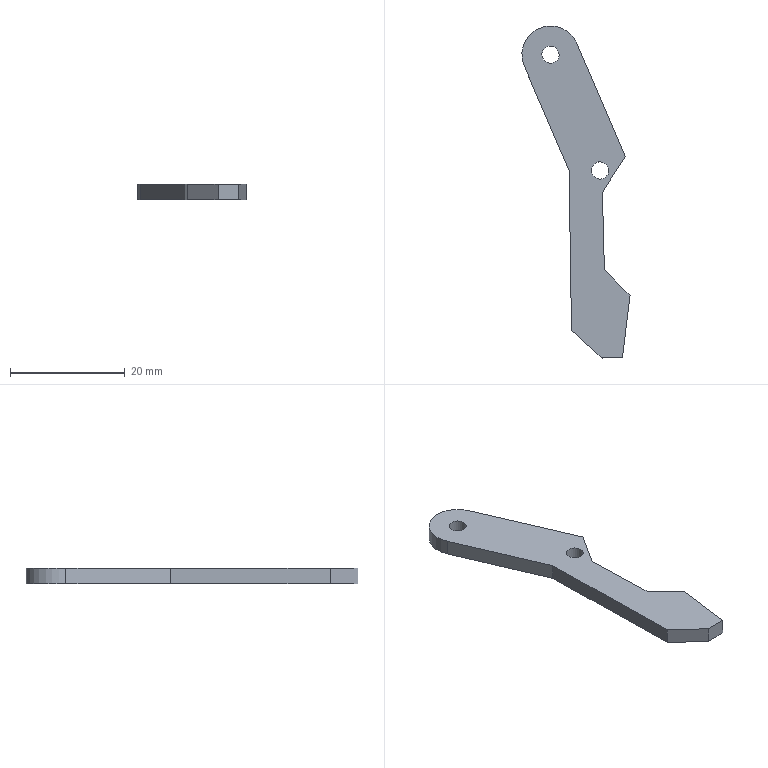Component | NX | GRIPPER_3 | 1 solid | 14 faces | box 18.88 x 57.93 x 2.7 mm | volume 1283 mm3 | plane 11 | cylinder 3 | commonest cylinder face diameters 3 x2 10 x1
STEP:
#1=CARTESIAN_POINT('',(0.,0.,0.));
#2=DIRECTION('',(0.,0.,1.));
#3=DIRECTION('',(1.,0.,0.));
#4=AXIS2_PLACEMENT_3D('',#1,#2,#3);
#5=CARTESIAN_POINT('',(-5.132,-91.783,35.05));
#6=VERTEX_POINT('',#5);
#7=CARTESIAN_POINT('',(-8.684,-91.838,35.05));
#8=VERTEX_POINT('',#7);
#9=CARTESIAN_POINT('',(-5.132,-91.783,35.05));
#10=DIRECTION('',(-0.9999,-0.01539,0.));
#11=VECTOR('',#10,1.);
#12=LINE('',#9,#11);
#13=CARTESIAN_POINT('',(-5.132,-91.783,32.35));
#14=DIRECTION('',(-0.01539,0.9999,0.));
#15=DIRECTION('',(-0.9999,-0.01539,0.));
#16=AXIS2_PLACEMENT_3D('',#13,#14,#15);
#17=PLANE('',#16);
#18=CARTESIAN_POINT('',(0.,2.7));
#19=DIRECTION('',(1.,0.));
#20=VECTOR('',#19,1.);
#21=LINE('',#18,#20);
#22=(GEOMETRIC_REPRESENTATION_CONTEXT(2)PARAMETRIC_REPRESENTATION_CONTEXT()REPRESENTATION_CONTEXT('',''));
#23=DEFINITIONAL_REPRESENTATION('',(#21),#22);
#24=PCURVE('',#17,#23);
#25=CARTESIAN_POINT('',(-17.683,-38.904,35.05));
#26=DIRECTION('',(0.,0.,-1.));
#27=DIRECTION('',(0.9189,0.3945,0.));
#28=AXIS2_PLACEMENT_3D('',#25,#26,#27);
#29=PLANE('',#28);
#30=CARTESIAN_POINT('',(-9.325,53.542));
#31=DIRECTION('',(-0.9249,-0.3803));
#32=VECTOR('',#31,1.);
#33=LINE('',#30,#32);
#34=(GEOMETRIC_REPRESENTATION_CONTEXT(2)PARAMETRIC_REPRESENTATION_CONTEXT()REPRESENTATION_CONTEXT('',''));
#35=DEFINITIONAL_REPRESENTATION('',(#33),#34);
#36=PCURVE('',#29,#35);
#37=SURFACE_CURVE('',#12,(#24,#36),.PCURVE_S1.);
#38=EDGE_CURVE('',#6,#8,#37,.T.);
#39=ORIENTED_EDGE('',*,*,#38,.T.);
#40=CARTESIAN_POINT('',(-8.684,-91.838,32.35));
#41=VERTEX_POINT('',#40);
#42=CARTESIAN_POINT('',(-8.684,-91.838,32.35));
#43=DIRECTION('',(0.,0.,1.));
#44=VECTOR('',#43,1.);
#45=LINE('',#42,#44);
#46=CARTESIAN_POINT('',(3.552,0.));
#47=DIRECTION('',(0.,1.));
#48=VECTOR('',#47,1.);
#49=LINE('',#46,#48);
#50=(GEOMETRIC_REPRESENTATION_CONTEXT(2)PARAMETRIC_REPRESENTATION_CONTEXT()REPRESENTATION_CONTEXT('',''));
#51=DEFINITIONAL_REPRESENTATION('',(#49),#50);
#52=PCURVE('',#17,#51);
#53=CARTESIAN_POINT('',(-8.684,-91.838,32.35));
#54=DIRECTION('',(0.6727,0.7399,0.));
#55=DIRECTION('',(-0.7399,0.6727,0.));
#56=AXIS2_PLACEMENT_3D('',#53,#54,#55);
#57=PLANE('',#56);
#58=CARTESIAN_POINT('',(0.,0.));
#59=DIRECTION('',(0.,1.));
#60=VECTOR('',#59,1.);
#61=LINE('',#58,#60);
#62=(GEOMETRIC_REPRESENTATION_CONTEXT(2)PARAMETRIC_REPRESENTATION_CONTEXT()REPRESENTATION_CONTEXT('',''));
#63=DEFINITIONAL_REPRESENTATION('',(#61),#62);
#64=PCURVE('',#57,#63);
#65=SURFACE_CURVE('',#45,(#52,#64),.PCURVE_S1.);
#66=EDGE_CURVE('',#41,#8,#65,.T.);
#67=ORIENTED_EDGE('',*,*,#66,.F.);
#68=CARTESIAN_POINT('',(-5.132,-91.783,32.35));
#69=VERTEX_POINT('',#68);
#70=CARTESIAN_POINT('',(-5.132,-91.783,32.35));
#71=DIRECTION('',(-0.9999,-0.01539,0.));
#72=VECTOR('',#71,1.);
#73=LINE('',#70,#72);
#74=CARTESIAN_POINT('',(0.,0.));
#75=DIRECTION('',(1.,0.));
#76=VECTOR('',#75,1.);
#77=LINE('',#74,#76);
#78=(GEOMETRIC_REPRESENTATION_CONTEXT(2)PARAMETRIC_REPRESENTATION_CONTEXT()REPRESENTATION_CONTEXT('',''));
#79=DEFINITIONAL_REPRESENTATION('',(#77),#78);
#80=PCURVE('',#17,#79);
#81=CARTESIAN_POINT('',(-17.683,-38.904,32.35));
#82=DIRECTION('',(0.,0.,-1.));
#83=DIRECTION('',(0.9189,0.3945,0.));
#84=AXIS2_PLACEMENT_3D('',#81,#82,#83);
#85=PLANE('',#84);
#86=CARTESIAN_POINT('',(-9.325,53.542));
#87=DIRECTION('',(-0.9249,-0.3803));
#88=VECTOR('',#87,1.);
#89=LINE('',#86,#88);
#90=(GEOMETRIC_REPRESENTATION_CONTEXT(2)PARAMETRIC_REPRESENTATION_CONTEXT()REPRESENTATION_CONTEXT('',''));
#91=DEFINITIONAL_REPRESENTATION('',(#89),#90);
#92=PCURVE('',#85,#91);
#93=SURFACE_CURVE('',#73,(#80,#92),.PCURVE_S1.);
#94=EDGE_CURVE('',#69,#41,#93,.T.);
#95=ORIENTED_EDGE('',*,*,#94,.F.);
#96=CARTESIAN_POINT('',(-5.132,-91.783,32.35));
#97=DIRECTION('',(0.,0.,1.));
#98=VECTOR('',#97,1.);
#99=LINE('',#96,#98);
#100=CARTESIAN_POINT('',(0.,0.));
#101=DIRECTION('',(0.,1.));
#102=VECTOR('',#101,1.);
#103=LINE('',#100,#102);
#104=(GEOMETRIC_REPRESENTATION_CONTEXT(2)PARAMETRIC_REPRESENTATION_CONTEXT()REPRESENTATION_CONTEXT('',''));
#105=DEFINITIONAL_REPRESENTATION('',(#103),#104);
#106=PCURVE('',#17,#105);
#107=CARTESIAN_POINT('',(-3.8,-80.896,32.35));
#108=DIRECTION('',(-0.9926,0.1214,0.));
#109=DIRECTION('',(-0.1214,-0.9926,0.));
#110=AXIS2_PLACEMENT_3D('',#107,#108,#109);
#111=PLANE('',#110);
#112=CARTESIAN_POINT('',(10.969,0.));
#113=DIRECTION('',(0.,1.));
#114=VECTOR('',#113,1.);
#115=LINE('',#112,#114);
#116=(GEOMETRIC_REPRESENTATION_CONTEXT(2)PARAMETRIC_REPRESENTATION_CONTEXT()REPRESENTATION_CONTEXT('',''));
#117=DEFINITIONAL_REPRESENTATION('',(#115),#116);
#118=PCURVE('',#111,#117);
#119=SURFACE_CURVE('',#99,(#106,#118),.PCURVE_S1.);
#120=EDGE_CURVE('',#69,#6,#119,.T.);
#121=ORIENTED_EDGE('',*,*,#120,.T.);
#122=EDGE_LOOP('',(#39,#67,#95,#121));
#123=FACE_BOUND('',#122,.T.);
#124=ADVANCED_FACE('',(#123),#17,.F.);
#125=CARTESIAN_POINT('',(-14.019,-86.988,35.05));
#126=VERTEX_POINT('',#125);
#127=CARTESIAN_POINT('',(-8.684,-91.838,35.05));
#128=DIRECTION('',(-0.7399,0.6727,0.));
#129=VECTOR('',#128,1.);
#130=LINE('',#127,#129);
#131=CARTESIAN_POINT('',(0.,2.7));
#132=DIRECTION('',(1.,0.));
#133=VECTOR('',#132,1.);
#134=LINE('',#131,#133);
#135=(GEOMETRIC_REPRESENTATION_CONTEXT(2)PARAMETRIC_REPRESENTATION_CONTEXT()REPRESENTATION_CONTEXT('',''));
#136=DEFINITIONAL_REPRESENTATION('',(#134),#135);
#137=PCURVE('',#57,#136);
#138=CARTESIAN_POINT('',(-12.611,52.191));
#139=DIRECTION('',(-0.4145,-0.91));
#140=VECTOR('',#139,1.);
#141=LINE('',#138,#140);
#142=(GEOMETRIC_REPRESENTATION_CONTEXT(2)PARAMETRIC_REPRESENTATION_CONTEXT()REPRESENTATION_CONTEXT('',''));
#143=DEFINITIONAL_REPRESENTATION('',(#141),#142);
#144=PCURVE('',#29,#143);
#145=SURFACE_CURVE('',#130,(#137,#144),.PCURVE_S1.);
#146=EDGE_CURVE('',#8,#126,#145,.T.);
#147=ORIENTED_EDGE('',*,*,#146,.T.);
#148=CARTESIAN_POINT('',(-14.019,-86.988,32.35));
#149=VERTEX_POINT('',#148);
#150=CARTESIAN_POINT('',(-14.019,-86.988,32.35));
#151=DIRECTION('',(0.,0.,1.));
#152=VECTOR('',#151,1.);
#153=LINE('',#150,#152);
#154=CARTESIAN_POINT('',(7.21,0.));
#155=DIRECTION('',(0.,1.));
#156=VECTOR('',#155,1.);
#157=LINE('',#154,#156);
#158=(GEOMETRIC_REPRESENTATION_CONTEXT(2)PARAMETRIC_REPRESENTATION_CONTEXT()REPRESENTATION_CONTEXT('',''));
#159=DEFINITIONAL_REPRESENTATION('',(#157),#158);
#160=PCURVE('',#57,#159);
#161=CARTESIAN_POINT('',(-14.019,-86.988,32.35));
#162=DIRECTION('',(0.9999,0.01539,0.));
#163=DIRECTION('',(-0.01539,0.9999,0.));
#164=AXIS2_PLACEMENT_3D('',#161,#162,#163);
#165=PLANE('',#164);
#166=CARTESIAN_POINT('',(0.,0.));
#167=DIRECTION('',(0.,1.));
#168=VECTOR('',#167,1.);
#169=LINE('',#166,#168);
#170=(GEOMETRIC_REPRESENTATION_CONTEXT(2)PARAMETRIC_REPRESENTATION_CONTEXT()REPRESENTATION_CONTEXT('',''));
#171=DEFINITIONAL_REPRESENTATION('',(#169),#170);
#172=PCURVE('',#165,#171);
#173=SURFACE_CURVE('',#153,(#160,#172),.PCURVE_S1.);
#174=EDGE_CURVE('',#149,#126,#173,.T.);
#175=ORIENTED_EDGE('',*,*,#174,.F.);
#176=CARTESIAN_POINT('',(-8.684,-91.838,32.35));
#177=DIRECTION('',(-0.7399,0.6727,0.));
#178=VECTOR('',#177,1.);
#179=LINE('',#176,#178);
#180=CARTESIAN_POINT('',(0.,0.));
#181=DIRECTION('',(1.,0.));
#182=VECTOR('',#181,1.);
#183=LINE('',#180,#182);
#184=(GEOMETRIC_REPRESENTATION_CONTEXT(2)PARAMETRIC_REPRESENTATION_CONTEXT()REPRESENTATION_CONTEXT('',''));
#185=DEFINITIONAL_REPRESENTATION('',(#183),#184);
#186=PCURVE('',#57,#185);
#187=CARTESIAN_POINT('',(-12.611,52.191));
#188=DIRECTION('',(-0.4145,-0.91));
#189=VECTOR('',#188,1.);
#190=LINE('',#187,#189);
#191=(GEOMETRIC_REPRESENTATION_CONTEXT(2)PARAMETRIC_REPRESENTATION_CONTEXT()REPRESENTATION_CONTEXT('',''));
#192=DEFINITIONAL_REPRESENTATION('',(#190),#191);
#193=PCURVE('',#85,#192);
#194=SURFACE_CURVE('',#179,(#186,#193),.PCURVE_S1.);
#195=EDGE_CURVE('',#41,#149,#194,.T.);
#196=ORIENTED_EDGE('',*,*,#195,.F.);
#197=ORIENTED_EDGE('',*,*,#66,.T.);
#198=EDGE_LOOP('',(#147,#175,#196,#197));
#199=FACE_BOUND('',#198,.T.);
#200=ADVANCED_FACE('',(#199),#57,.F.);
#201=CARTESIAN_POINT('',(-14.448,-59.117,35.05));
#202=VERTEX_POINT('',#201);
#203=CARTESIAN_POINT('',(-14.019,-86.988,35.05));
#204=DIRECTION('',(-0.01539,0.9999,0.));
#205=VECTOR('',#204,1.);
#206=LINE('',#203,#205);
#207=CARTESIAN_POINT('',(0.,2.7));
#208=DIRECTION('',(1.,0.));
#209=VECTOR('',#208,1.);
#210=LINE('',#207,#209);
#211=(GEOMETRIC_REPRESENTATION_CONTEXT(2)PARAMETRIC_REPRESENTATION_CONTEXT()REPRESENTATION_CONTEXT('',''));
#212=DEFINITIONAL_REPRESENTATION('',(#210),#211);
#213=PCURVE('',#165,#212);
#214=CARTESIAN_POINT('',(-15.599,45.63));
#215=DIRECTION('',(0.3803,-0.9249));
#216=VECTOR('',#215,1.);
#217=LINE('',#214,#216);
#218=(GEOMETRIC_REPRESENTATION_CONTEXT(2)PARAMETRIC_REPRESENTATION_CONTEXT()REPRESENTATION_CONTEXT('',''));
#219=DEFINITIONAL_REPRESENTATION('',(#217),#218);
#220=PCURVE('',#29,#219);
#221=SURFACE_CURVE('',#206,(#213,#220),.PCURVE_S1.);
#222=EDGE_CURVE('',#126,#202,#221,.T.);
#223=ORIENTED_EDGE('',*,*,#222,.T.);
#224=CARTESIAN_POINT('',(-14.448,-59.117,32.35));
#225=VERTEX_POINT('',#224);
#226=CARTESIAN_POINT('',(-14.448,-59.117,32.35));
#227=DIRECTION('',(0.,0.,1.));
#228=VECTOR('',#227,1.);
#229=LINE('',#226,#228);
#230=CARTESIAN_POINT('',(27.874,0.));
#231=DIRECTION('',(0.,1.));
#232=VECTOR('',#231,1.);
#233=LINE('',#230,#232);
#234=(GEOMETRIC_REPRESENTATION_CONTEXT(2)PARAMETRIC_REPRESENTATION_CONTEXT()REPRESENTATION_CONTEXT('',''));
#235=DEFINITIONAL_REPRESENTATION('',(#233),#234);
#236=PCURVE('',#165,#235);
#237=CARTESIAN_POINT('',(-14.448,-59.117,32.35));
#238=DIRECTION('',(0.9189,0.3945,0.));
#239=DIRECTION('',(-0.3945,0.9189,0.));
#240=AXIS2_PLACEMENT_3D('',#237,#238,#239);
#241=PLANE('',#240);
#242=CARTESIAN_POINT('',(0.,0.));
#243=DIRECTION('',(0.,1.));
#244=VECTOR('',#243,1.);
#245=LINE('',#242,#244);
#246=(GEOMETRIC_REPRESENTATION_CONTEXT(2)PARAMETRIC_REPRESENTATION_CONTEXT()REPRESENTATION_CONTEXT('',''));
#247=DEFINITIONAL_REPRESENTATION('',(#245),#246);
#248=PCURVE('',#241,#247);
#249=SURFACE_CURVE('',#229,(#236,#248),.PCURVE_S1.);
#250=EDGE_CURVE('',#225,#202,#249,.T.);
#251=ORIENTED_EDGE('',*,*,#250,.F.);
#252=CARTESIAN_POINT('',(-14.019,-86.988,32.35));
#253=DIRECTION('',(-0.01539,0.9999,0.));
#254=VECTOR('',#253,1.);
#255=LINE('',#252,#254);
#256=CARTESIAN_POINT('',(0.,0.));
#257=DIRECTION('',(1.,0.));
#258=VECTOR('',#257,1.);
#259=LINE('',#256,#258);
#260=(GEOMETRIC_REPRESENTATION_CONTEXT(2)PARAMETRIC_REPRESENTATION_CONTEXT()REPRESENTATION_CONTEXT('',''));
#261=DEFINITIONAL_REPRESENTATION('',(#259),#260);
#262=PCURVE('',#165,#261);
#263=CARTESIAN_POINT('',(-15.599,45.63));
#264=DIRECTION('',(0.3803,-0.9249));
#265=VECTOR('',#264,1.);
#266=LINE('',#263,#265);
#267=(GEOMETRIC_REPRESENTATION_CONTEXT(2)PARAMETRIC_REPRESENTATION_CONTEXT()REPRESENTATION_CONTEXT('',''));
#268=DEFINITIONAL_REPRESENTATION('',(#266),#267);
#269=PCURVE('',#85,#268);
#270=SURFACE_CURVE('',#255,(#262,#269),.PCURVE_S1.);
#271=EDGE_CURVE('',#149,#225,#270,.T.);
#272=ORIENTED_EDGE('',*,*,#271,.F.);
#273=ORIENTED_EDGE('',*,*,#174,.T.);
#274=EDGE_LOOP('',(#223,#251,#272,#273));
#275=FACE_BOUND('',#274,.T.);
#276=ADVANCED_FACE('',(#275),#165,.F.);
#277=CARTESIAN_POINT('',(-22.278,-40.877,35.05));
#278=VERTEX_POINT('',#277);
#279=CARTESIAN_POINT('',(-14.448,-59.117,35.05));
#280=DIRECTION('',(-0.3945,0.9189,0.));
#281=VECTOR('',#280,1.);
#282=LINE('',#279,#281);
#283=CARTESIAN_POINT('',(0.,2.7));
#284=DIRECTION('',(1.,0.));
#285=VECTOR('',#284,1.);
#286=LINE('',#283,#285);
#287=(GEOMETRIC_REPRESENTATION_CONTEXT(2)PARAMETRIC_REPRESENTATION_CONTEXT()REPRESENTATION_CONTEXT('',''));
#288=DEFINITIONAL_REPRESENTATION('',(#286),#287);
#289=PCURVE('',#241,#288);
#290=CARTESIAN_POINT('',(-5.,19.85));
#291=DIRECTION('',(0.,-1.));
#292=VECTOR('',#291,1.);
#293=LINE('',#290,#292);
#294=(GEOMETRIC_REPRESENTATION_CONTEXT(2)PARAMETRIC_REPRESENTATION_CONTEXT()REPRESENTATION_CONTEXT('',''));
#295=DEFINITIONAL_REPRESENTATION('',(#293),#294);
#296=PCURVE('',#29,#295);
#297=SURFACE_CURVE('',#282,(#289,#296),.PCURVE_S1.);
#298=EDGE_CURVE('',#202,#278,#297,.T.);
#299=ORIENTED_EDGE('',*,*,#298,.T.);
#300=CARTESIAN_POINT('',(-22.278,-40.877,32.35));
#301=VERTEX_POINT('',#300);
#302=CARTESIAN_POINT('',(-22.278,-40.877,32.35));
#303=DIRECTION('',(0.,0.,1.));
#304=VECTOR('',#303,1.);
#305=LINE('',#302,#304);
#306=CARTESIAN_POINT('',(19.85,0.));
#307=DIRECTION('',(0.,1.));
#308=VECTOR('',#307,1.);
#309=LINE('',#306,#308);
#310=(GEOMETRIC_REPRESENTATION_CONTEXT(2)PARAMETRIC_REPRESENTATION_CONTEXT()REPRESENTATION_CONTEXT('',''));
#311=DEFINITIONAL_REPRESENTATION('',(#309),#310);
#312=PCURVE('',#241,#311);
#313=CARTESIAN_POINT('',(-17.683,-38.904,32.35));
#314=DIRECTION('',(0.,0.,1.));
#315=DIRECTION('',(-0.9189,-0.3945,0.));
#316=AXIS2_PLACEMENT_3D('',#313,#314,#315);
#317=CYLINDRICAL_SURFACE('',#316,5.);
#318=CARTESIAN_POINT('',(6.283,0.));
#319=DIRECTION('',(0.,1.));
#320=VECTOR('',#319,1.);
#321=LINE('',#318,#320);
#322=(GEOMETRIC_REPRESENTATION_CONTEXT(2)PARAMETRIC_REPRESENTATION_CONTEXT()REPRESENTATION_CONTEXT('',''));
#323=DEFINITIONAL_REPRESENTATION('',(#321),#322);
#324=PCURVE('',#317,#323);
#325=SURFACE_CURVE('',#305,(#312,#324),.PCURVE_S1.);
#326=EDGE_CURVE('',#301,#278,#325,.T.);
#327=ORIENTED_EDGE('',*,*,#326,.F.);
#328=CARTESIAN_POINT('',(-14.448,-59.117,32.35));
#329=DIRECTION('',(-0.3945,0.9189,0.));
#330=VECTOR('',#329,1.);
#331=LINE('',#328,#330);
#332=CARTESIAN_POINT('',(0.,0.));
#333=DIRECTION('',(1.,0.));
#334=VECTOR('',#333,1.);
#335=LINE('',#332,#334);
#336=(GEOMETRIC_REPRESENTATION_CONTEXT(2)PARAMETRIC_REPRESENTATION_CONTEXT()REPRESENTATION_CONTEXT('',''));
#337=DEFINITIONAL_REPRESENTATION('',(#335),#336);
#338=PCURVE('',#241,#337);
#339=CARTESIAN_POINT('',(-5.,19.85));
#340=DIRECTION('',(0.,-1.));
#341=VECTOR('',#340,1.);
#342=LINE('',#339,#341);
#343=(GEOMETRIC_REPRESENTATION_CONTEXT(2)PARAMETRIC_REPRESENTATION_CONTEXT()REPRESENTATION_CONTEXT('',''));
#344=DEFINITIONAL_REPRESENTATION('',(#342),#343);
#345=PCURVE('',#85,#344);
#346=SURFACE_CURVE('',#331,(#338,#345),.PCURVE_S1.);
#347=EDGE_CURVE('',#225,#301,#346,.T.);
#348=ORIENTED_EDGE('',*,*,#347,.F.);
#349=ORIENTED_EDGE('',*,*,#250,.T.);
#350=EDGE_LOOP('',(#299,#327,#348,#349));
#351=FACE_BOUND('',#350,.T.);
#352=ADVANCED_FACE('',(#351),#241,.F.);
#353=CARTESIAN_POINT('',(-13.088,-36.932,35.05));
#354=VERTEX_POINT('',#353);
#355=CARTESIAN_POINT('',(-17.683,-38.904,35.05));
#356=DIRECTION('',(0.,0.,-1.));
#357=DIRECTION('',(0.3945,-0.9189,0.));
#358=AXIS2_PLACEMENT_3D('',#355,#356,#357);
#359=CIRCLE('',#358,5.);
#360=CARTESIAN_POINT('',(7.854,2.7));
#361=DIRECTION('',(-1.,0.));
#362=VECTOR('',#361,1.);
#363=LINE('',#360,#362);
#364=(GEOMETRIC_REPRESENTATION_CONTEXT(2)PARAMETRIC_REPRESENTATION_CONTEXT()REPRESENTATION_CONTEXT('',''));
#365=DEFINITIONAL_REPRESENTATION('',(#363),#364);
#366=PCURVE('',#317,#365);
#367=CARTESIAN_POINT('',(0.,0.));
#368=DIRECTION('',(0.,1.));
#369=AXIS2_PLACEMENT_2D('',#367,#368);
#370=CIRCLE('',#369,5.);
#371=(GEOMETRIC_REPRESENTATION_CONTEXT(2)PARAMETRIC_REPRESENTATION_CONTEXT()REPRESENTATION_CONTEXT('',''));
#372=DEFINITIONAL_REPRESENTATION('',(#370),#371);
#373=PCURVE('',#29,#372);
#374=SURFACE_CURVE('',#359,(#366,#373),.PCURVE_S1.);
#375=EDGE_CURVE('',#278,#354,#374,.T.);
#376=ORIENTED_EDGE('',*,*,#375,.T.);
#377=CARTESIAN_POINT('',(-13.088,-36.932,32.35));
#378=VERTEX_POINT('',#377);
#379=CARTESIAN_POINT('',(-13.088,-36.932,32.35));
#380=DIRECTION('',(0.,0.,1.));
#381=VECTOR('',#380,1.);
#382=LINE('',#379,#381);
#383=CARTESIAN_POINT('',(3.142,0.));
#384=DIRECTION('',(0.,1.));
#385=VECTOR('',#384,1.);
#386=LINE('',#383,#385);
#387=(GEOMETRIC_REPRESENTATION_CONTEXT(2)PARAMETRIC_REPRESENTATION_CONTEXT()REPRESENTATION_CONTEXT('',''));
#388=DEFINITIONAL_REPRESENTATION('',(#386),#387);
#389=PCURVE('',#317,#388);
#390=CARTESIAN_POINT('',(-13.088,-36.932,32.35));
#391=DIRECTION('',(-0.9189,-0.3945,0.));
#392=DIRECTION('',(0.3945,-0.9189,0.));
#393=AXIS2_PLACEMENT_3D('',#390,#391,#392);
#394=PLANE('',#393);
#395=CARTESIAN_POINT('',(0.,0.));
#396=DIRECTION('',(0.,1.));
#397=VECTOR('',#396,1.);
#398=LINE('',#395,#397);
#399=(GEOMETRIC_REPRESENTATION_CONTEXT(2)PARAMETRIC_REPRESENTATION_CONTEXT()REPRESENTATION_CONTEXT('',''));
#400=DEFINITIONAL_REPRESENTATION('',(#398),#399);
#401=PCURVE('',#394,#400);
#402=SURFACE_CURVE('',#382,(#389,#401),.PCURVE_S1.);
#403=EDGE_CURVE('',#378,#354,#402,.T.);
#404=ORIENTED_EDGE('',*,*,#403,.F.);
#405=CARTESIAN_POINT('',(-17.683,-38.904,32.35));
#406=DIRECTION('',(0.,0.,-1.));
#407=DIRECTION('',(0.3945,-0.9189,0.));
#408=AXIS2_PLACEMENT_3D('',#405,#406,#407);
#409=CIRCLE('',#408,5.);
#410=CARTESIAN_POINT('',(7.854,0.));
#411=DIRECTION('',(-1.,0.));
#412=VECTOR('',#411,1.);
#413=LINE('',#410,#412);
#414=(GEOMETRIC_REPRESENTATION_CONTEXT(2)PARAMETRIC_REPRESENTATION_CONTEXT()REPRESENTATION_CONTEXT('',''));
#415=DEFINITIONAL_REPRESENTATION('',(#413),#414);
#416=PCURVE('',#317,#415);
#417=CARTESIAN_POINT('',(0.,0.));
#418=DIRECTION('',(0.,1.));
#419=AXIS2_PLACEMENT_2D('',#417,#418);
#420=CIRCLE('',#419,5.);
#421=(GEOMETRIC_REPRESENTATION_CONTEXT(2)PARAMETRIC_REPRESENTATION_CONTEXT()REPRESENTATION_CONTEXT('',''));
#422=DEFINITIONAL_REPRESENTATION('',(#420),#421);
#423=PCURVE('',#85,#422);
#424=SURFACE_CURVE('',#409,(#416,#423),.PCURVE_S1.);
#425=EDGE_CURVE('',#301,#378,#424,.T.);
#426=ORIENTED_EDGE('',*,*,#425,.F.);
#427=ORIENTED_EDGE('',*,*,#326,.T.);
#428=EDGE_LOOP('',(#376,#404,#426,#427));
#429=FACE_BOUND('',#428,.T.);
#430=ADVANCED_FACE('',(#429),#317,.T.);
#431=CARTESIAN_POINT('',(-4.62,-56.661,35.05));
#432=VERTEX_POINT('',#431);
#433=CARTESIAN_POINT('',(-13.088,-36.932,35.05));
#434=DIRECTION('',(0.3945,-0.9189,0.));
#435=VECTOR('',#434,1.);
#436=LINE('',#433,#435);
#437=CARTESIAN_POINT('',(0.,2.7));
#438=DIRECTION('',(1.,0.));
#439=VECTOR('',#438,1.);
#440=LINE('',#437,#439);
#441=(GEOMETRIC_REPRESENTATION_CONTEXT(2)PARAMETRIC_REPRESENTATION_CONTEXT()REPRESENTATION_CONTEXT('',''));
#442=DEFINITIONAL_REPRESENTATION('',(#440),#441);
#443=PCURVE('',#394,#442);
#444=CARTESIAN_POINT('',(5.,0.));
#445=DIRECTION('',(0.,1.));
#446=VECTOR('',#445,1.);
#447=LINE('',#444,#446);
#448=(GEOMETRIC_REPRESENTATION_CONTEXT(2)PARAMETRIC_REPRESENTATION_CONTEXT()REPRESENTATION_CONTEXT('',''));
#449=DEFINITIONAL_REPRESENTATION('',(#447),#448);
#450=PCURVE('',#29,#449);
#451=SURFACE_CURVE('',#436,(#443,#450),.PCURVE_S1.);
#452=EDGE_CURVE('',#354,#432,#451,.T.);
#453=ORIENTED_EDGE('',*,*,#452,.T.);
#454=CARTESIAN_POINT('',(-4.62,-56.661,32.35));
#455=VERTEX_POINT('',#454);
#456=CARTESIAN_POINT('',(-4.62,-56.661,32.35));
#457=DIRECTION('',(0.,0.,1.));
#458=VECTOR('',#457,1.);
#459=LINE('',#456,#458);
#460=CARTESIAN_POINT('',(21.47,0.));
#461=DIRECTION('',(0.,1.));
#462=VECTOR('',#461,1.);
#463=LINE('',#460,#462);
#464=(GEOMETRIC_REPRESENTATION_CONTEXT(2)PARAMETRIC_REPRESENTATION_CONTEXT()REPRESENTATION_CONTEXT('',''));
#465=DEFINITIONAL_REPRESENTATION('',(#463),#464);
#466=PCURVE('',#394,#465);
#467=CARTESIAN_POINT('',(-4.62,-56.661,32.35));
#468=DIRECTION('',(-0.8421,0.5393,0.));
#469=DIRECTION('',(-0.5393,-0.8421,0.));
#470=AXIS2_PLACEMENT_3D('',#467,#468,#469);
#471=PLANE('',#470);
#472=CARTESIAN_POINT('',(0.,0.));
#473=DIRECTION('',(0.,1.));
#474=VECTOR('',#473,1.);
#475=LINE('',#472,#474);
#476=(GEOMETRIC_REPRESENTATION_CONTEXT(2)PARAMETRIC_REPRESENTATION_CONTEXT()REPRESENTATION_CONTEXT('',''));
#477=DEFINITIONAL_REPRESENTATION('',(#475),#476);
#478=PCURVE('',#471,#477);
#479=SURFACE_CURVE('',#459,(#466,#478),.PCURVE_S1.);
#480=EDGE_CURVE('',#455,#432,#479,.T.);
#481=ORIENTED_EDGE('',*,*,#480,.F.);
#482=CARTESIAN_POINT('',(-13.088,-36.932,32.35));
#483=DIRECTION('',(0.3945,-0.9189,0.));
#484=VECTOR('',#483,1.);
#485=LINE('',#482,#484);
#486=CARTESIAN_POINT('',(0.,0.));
#487=DIRECTION('',(1.,0.));
#488=VECTOR('',#487,1.);
#489=LINE('',#486,#488);
#490=(GEOMETRIC_REPRESENTATION_CONTEXT(2)PARAMETRIC_REPRESENTATION_CONTEXT()REPRESENTATION_CONTEXT('',''));
#491=DEFINITIONAL_REPRESENTATION('',(#489),#490);
#492=PCURVE('',#394,#491);
#493=CARTESIAN_POINT('',(5.,0.));
#494=DIRECTION('',(0.,1.));
#495=VECTOR('',#494,1.);
#496=LINE('',#493,#495);
#497=(GEOMETRIC_REPRESENTATION_CONTEXT(2)PARAMETRIC_REPRESENTATION_CONTEXT()REPRESENTATION_CONTEXT('',''));
#498=DEFINITIONAL_REPRESENTATION('',(#496),#497);
#499=PCURVE('',#85,#498);
#500=SURFACE_CURVE('',#485,(#492,#499),.PCURVE_S1.);
#501=EDGE_CURVE('',#378,#455,#500,.T.);
#502=ORIENTED_EDGE('',*,*,#501,.F.);
#503=ORIENTED_EDGE('',*,*,#403,.T.);
#504=EDGE_LOOP('',(#453,#481,#502,#503));
#505=FACE_BOUND('',#504,.T.);
#506=ADVANCED_FACE('',(#505),#394,.F.);
#507=CARTESIAN_POINT('',(-8.632,-62.926,35.05));
#508=VERTEX_POINT('',#507);
#509=CARTESIAN_POINT('',(-4.62,-56.661,35.05));
#510=DIRECTION('',(-0.5393,-0.8421,0.));
#511=VECTOR('',#510,1.);
#512=LINE('',#509,#511);
#513=CARTESIAN_POINT('',(0.,2.7));
#514=DIRECTION('',(1.,0.));
#515=VECTOR('',#514,1.);
#516=LINE('',#513,#515);
#517=(GEOMETRIC_REPRESENTATION_CONTEXT(2)PARAMETRIC_REPRESENTATION_CONTEXT()REPRESENTATION_CONTEXT('',''));
#518=DEFINITIONAL_REPRESENTATION('',(#516),#517);
#519=PCURVE('',#471,#518);
#520=CARTESIAN_POINT('',(5.,21.47));
#521=DIRECTION('',(-0.8278,0.5611));
#522=VECTOR('',#521,1.);
#523=LINE('',#520,#522);
#524=(GEOMETRIC_REPRESENTATION_CONTEXT(2)PARAMETRIC_REPRESENTATION_CONTEXT()REPRESENTATION_CONTEXT('',''));
#525=DEFINITIONAL_REPRESENTATION('',(#523),#524);
#526=PCURVE('',#29,#525);
#527=SURFACE_CURVE('',#512,(#519,#526),.PCURVE_S1.);
#528=EDGE_CURVE('',#432,#508,#527,.T.);
#529=ORIENTED_EDGE('',*,*,#528,.T.);
#530=CARTESIAN_POINT('',(-8.632,-62.926,32.35));
#531=VERTEX_POINT('',#530);
#532=CARTESIAN_POINT('',(-8.632,-62.926,32.35));
#533=DIRECTION('',(0.,0.,1.));
#534=VECTOR('',#533,1.);
#535=LINE('',#532,#534);
#536=CARTESIAN_POINT('',(7.44,0.));
#537=DIRECTION('',(0.,1.));
#538=VECTOR('',#537,1.);
#539=LINE('',#536,#538);
#540=(GEOMETRIC_REPRESENTATION_CONTEXT(2)PARAMETRIC_REPRESENTATION_CONTEXT()REPRESENTATION_CONTEXT('',''));
#541=DEFINITIONAL_REPRESENTATION('',(#539),#540);
#542=PCURVE('',#471,#541);
#543=CARTESIAN_POINT('',(-8.632,-62.926,32.35));
#544=DIRECTION('',(-0.9997,-0.02603,0.));
#545=DIRECTION('',(0.02603,-0.9997,0.));
#546=AXIS2_PLACEMENT_3D('',#543,#544,#545);
#547=PLANE('',#546);
#548=CARTESIAN_POINT('',(0.,0.));
#549=DIRECTION('',(0.,1.));
#550=VECTOR('',#549,1.);
#551=LINE('',#548,#550);
#552=(GEOMETRIC_REPRESENTATION_CONTEXT(2)PARAMETRIC_REPRESENTATION_CONTEXT()REPRESENTATION_CONTEXT('',''));
#553=DEFINITIONAL_REPRESENTATION('',(#551),#552);
#554=PCURVE('',#547,#553);
#555=SURFACE_CURVE('',#535,(#542,#554),.PCURVE_S1.);
#556=EDGE_CURVE('',#531,#508,#555,.T.);
#557=ORIENTED_EDGE('',*,*,#556,.F.);
#558=CARTESIAN_POINT('',(-4.62,-56.661,32.35));
#559=DIRECTION('',(-0.5393,-0.8421,0.));
#560=VECTOR('',#559,1.);
#561=LINE('',#558,#560);
#562=CARTESIAN_POINT('',(0.,0.));
#563=DIRECTION('',(1.,0.));
#564=VECTOR('',#563,1.);
#565=LINE('',#562,#564);
#566=(GEOMETRIC_REPRESENTATION_CONTEXT(2)PARAMETRIC_REPRESENTATION_CONTEXT()REPRESENTATION_CONTEXT('',''));
#567=DEFINITIONAL_REPRESENTATION('',(#565),#566);
#568=PCURVE('',#471,#567);
#569=CARTESIAN_POINT('',(5.,21.47));
#570=DIRECTION('',(-0.8278,0.5611));
#571=VECTOR('',#570,1.);
#572=LINE('',#569,#571);
#573=(GEOMETRIC_REPRESENTATION_CONTEXT(2)PARAMETRIC_REPRESENTATION_CONTEXT()REPRESENTATION_CONTEXT('',''));
#574=DEFINITIONAL_REPRESENTATION('',(#572),#573);
#575=PCURVE('',#85,#574);
#576=SURFACE_CURVE('',#561,(#568,#575),.PCURVE_S1.);
#577=EDGE_CURVE('',#455,#531,#576,.T.);
#578=ORIENTED_EDGE('',*,*,#577,.F.);
#579=ORIENTED_EDGE('',*,*,#480,.T.);
#580=EDGE_LOOP('',(#529,#557,#578,#579));
#581=FACE_BOUND('',#580,.T.);
#582=ADVANCED_FACE('',(#581),#471,.F.);
#583=CARTESIAN_POINT('',(-8.28,-76.452,35.05));
#584=VERTEX_POINT('',#583);
#585=CARTESIAN_POINT('',(-8.632,-62.926,35.05));
#586=DIRECTION('',(0.02603,-0.9997,0.));
#587=VECTOR('',#586,1.);
#588=LINE('',#585,#587);
#589=CARTESIAN_POINT('',(0.,2.7));
#590=DIRECTION('',(1.,0.));
#591=VECTOR('',#590,1.);
#592=LINE('',#589,#591);
#593=(GEOMETRIC_REPRESENTATION_CONTEXT(2)PARAMETRIC_REPRESENTATION_CONTEXT()REPRESENTATION_CONTEXT('',''));
#594=DEFINITIONAL_REPRESENTATION('',(#592),#593);
#595=PCURVE('',#547,#594);
#596=CARTESIAN_POINT('',(-1.159,25.644));
#597=DIRECTION('',(-0.3704,0.9289));
#598=VECTOR('',#597,1.);
#599=LINE('',#596,#598);
#600=(GEOMETRIC_REPRESENTATION_CONTEXT(2)PARAMETRIC_REPRESENTATION_CONTEXT()REPRESENTATION_CONTEXT('',''));
#601=DEFINITIONAL_REPRESENTATION('',(#599),#600);
#602=PCURVE('',#29,#601);
#603=SURFACE_CURVE('',#588,(#595,#602),.PCURVE_S1.);
#604=EDGE_CURVE('',#508,#584,#603,.T.);
#605=ORIENTED_EDGE('',*,*,#604,.T.);
#606=CARTESIAN_POINT('',(-8.28,-76.452,32.35));
#607=VERTEX_POINT('',#606);
#608=CARTESIAN_POINT('',(-8.28,-76.452,32.35));
#609=DIRECTION('',(0.,0.,1.));
#610=VECTOR('',#609,1.);
#611=LINE('',#608,#610);
#612=CARTESIAN_POINT('',(13.53,0.));
#613=DIRECTION('',(0.,1.));
#614=VECTOR('',#613,1.);
#615=LINE('',#612,#614);
#616=(GEOMETRIC_REPRESENTATION_CONTEXT(2)PARAMETRIC_REPRESENTATION_CONTEXT()REPRESENTATION_CONTEXT('',''));
#617=DEFINITIONAL_REPRESENTATION('',(#615),#616);
#618=PCURVE('',#547,#617);
#619=CARTESIAN_POINT('',(-8.28,-76.452,32.35));
#620=DIRECTION('',(-0.7042,-0.71,0.));
#621=DIRECTION('',(0.71,-0.7042,0.));
#622=AXIS2_PLACEMENT_3D('',#619,#620,#621);
#623=PLANE('',#622);
#624=CARTESIAN_POINT('',(0.,0.));
#625=DIRECTION('',(0.,1.));
#626=VECTOR('',#625,1.);
#627=LINE('',#624,#626);
#628=(GEOMETRIC_REPRESENTATION_CONTEXT(2)PARAMETRIC_REPRESENTATION_CONTEXT()REPRESENTATION_CONTEXT('',''));
#629=DEFINITIONAL_REPRESENTATION('',(#627),#628);
#630=PCURVE('',#623,#629);
#631=SURFACE_CURVE('',#611,(#618,#630),.PCURVE_S1.);
#632=EDGE_CURVE('',#607,#584,#631,.T.);
#633=ORIENTED_EDGE('',*,*,#632,.F.);
#634=CARTESIAN_POINT('',(-8.632,-62.926,32.35));
#635=DIRECTION('',(0.02603,-0.9997,0.));
#636=VECTOR('',#635,1.);
#637=LINE('',#634,#636);
#638=CARTESIAN_POINT('',(0.,0.));
#639=DIRECTION('',(1.,0.));
#640=VECTOR('',#639,1.);
#641=LINE('',#638,#640);
#642=(GEOMETRIC_REPRESENTATION_CONTEXT(2)PARAMETRIC_REPRESENTATION_CONTEXT()REPRESENTATION_CONTEXT('',''));
#643=DEFINITIONAL_REPRESENTATION('',(#641),#642);
#644=PCURVE('',#547,#643);
#645=CARTESIAN_POINT('',(-1.159,25.644));
#646=DIRECTION('',(-0.3704,0.9289));
#647=VECTOR('',#646,1.);
#648=LINE('',#645,#647);
#649=(GEOMETRIC_REPRESENTATION_CONTEXT(2)PARAMETRIC_REPRESENTATION_CONTEXT()REPRESENTATION_CONTEXT('',''));
#650=DEFINITIONAL_REPRESENTATION('',(#648),#649);
#651=PCURVE('',#85,#650);
#652=SURFACE_CURVE('',#637,(#644,#651),.PCURVE_S1.);
#653=EDGE_CURVE('',#531,#607,#652,.T.);
#654=ORIENTED_EDGE('',*,*,#653,.F.);
#655=ORIENTED_EDGE('',*,*,#556,.T.);
#656=EDGE_LOOP('',(#605,#633,#654,#655));
#657=FACE_BOUND('',#656,.T.);
#658=ADVANCED_FACE('',(#657),#547,.F.);
#659=CARTESIAN_POINT('',(-3.8,-80.896,35.05));
#660=VERTEX_POINT('',#659);
#661=CARTESIAN_POINT('',(-8.28,-76.452,35.05));
#662=DIRECTION('',(0.71,-0.7042,0.));
#663=VECTOR('',#662,1.);
#664=LINE('',#661,#663);
#665=CARTESIAN_POINT('',(0.,2.7));
#666=DIRECTION('',(1.,0.));
#667=VECTOR('',#666,1.);
#668=LINE('',#665,#667);
#669=(GEOMETRIC_REPRESENTATION_CONTEXT(2)PARAMETRIC_REPRESENTATION_CONTEXT()REPRESENTATION_CONTEXT('',''));
#670=DEFINITIONAL_REPRESENTATION('',(#668),#669);
#671=PCURVE('',#623,#670);
#672=CARTESIAN_POINT('',(-6.17,38.212));
#673=DIRECTION('',(0.3746,0.9272));
#674=VECTOR('',#673,1.);
#675=LINE('',#672,#674);
#676=(GEOMETRIC_REPRESENTATION_CONTEXT(2)PARAMETRIC_REPRESENTATION_CONTEXT()REPRESENTATION_CONTEXT('',''));
#677=DEFINITIONAL_REPRESENTATION('',(#675),#676);
#678=PCURVE('',#29,#677);
#679=SURFACE_CURVE('',#664,(#671,#678),.PCURVE_S1.);
#680=EDGE_CURVE('',#584,#660,#679,.T.);
#681=ORIENTED_EDGE('',*,*,#680,.T.);
#682=CARTESIAN_POINT('',(-3.8,-80.896,32.35));
#683=VERTEX_POINT('',#682);
#684=CARTESIAN_POINT('',(-3.8,-80.896,32.35));
#685=DIRECTION('',(0.,0.,1.));
#686=VECTOR('',#685,1.);
#687=LINE('',#684,#686);
#688=CARTESIAN_POINT('',(6.31,0.));
#689=DIRECTION('',(0.,1.));
#690=VECTOR('',#689,1.);
#691=LINE('',#688,#690);
#692=(GEOMETRIC_REPRESENTATION_CONTEXT(2)PARAMETRIC_REPRESENTATION_CONTEXT()REPRESENTATION_CONTEXT('',''));
#693=DEFINITIONAL_REPRESENTATION('',(#691),#692);
#694=PCURVE('',#623,#693);
#695=CARTESIAN_POINT('',(0.,0.));
#696=DIRECTION('',(0.,1.));
#697=VECTOR('',#696,1.);
#698=LINE('',#695,#697);
#699=(GEOMETRIC_REPRESENTATION_CONTEXT(2)PARAMETRIC_REPRESENTATION_CONTEXT()REPRESENTATION_CONTEXT('',''));
#700=DEFINITIONAL_REPRESENTATION('',(#698),#699);
#701=PCURVE('',#111,#700);
#702=SURFACE_CURVE('',#687,(#694,#701),.PCURVE_S1.);
#703=EDGE_CURVE('',#683,#660,#702,.T.);
#704=ORIENTED_EDGE('',*,*,#703,.F.);
#705=CARTESIAN_POINT('',(-8.28,-76.452,32.35));
#706=DIRECTION('',(0.71,-0.7042,0.));
#707=VECTOR('',#706,1.);
#708=LINE('',#705,#707);
#709=CARTESIAN_POINT('',(0.,0.));
#710=DIRECTION('',(1.,0.));
#711=VECTOR('',#710,1.);
#712=LINE('',#709,#711);
#713=(GEOMETRIC_REPRESENTATION_CONTEXT(2)PARAMETRIC_REPRESENTATION_CONTEXT()REPRESENTATION_CONTEXT('',''));
#714=DEFINITIONAL_REPRESENTATION('',(#712),#713);
#715=PCURVE('',#623,#714);
#716=CARTESIAN_POINT('',(-6.17,38.212));
#717=DIRECTION('',(0.3746,0.9272));
#718=VECTOR('',#717,1.);
#719=LINE('',#716,#718);
#720=(GEOMETRIC_REPRESENTATION_CONTEXT(2)PARAMETRIC_REPRESENTATION_CONTEXT()REPRESENTATION_CONTEXT('',''));
#721=DEFINITIONAL_REPRESENTATION('',(#719),#720);
#722=PCURVE('',#85,#721);
#723=SURFACE_CURVE('',#708,(#715,#722),.PCURVE_S1.);
#724=EDGE_CURVE('',#607,#683,#723,.T.);
#725=ORIENTED_EDGE('',*,*,#724,.F.);
#726=ORIENTED_EDGE('',*,*,#632,.T.);
#727=EDGE_LOOP('',(#681,#704,#725,#726));
#728=FACE_BOUND('',#727,.T.);
#729=ADVANCED_FACE('',(#728),#623,.F.);
#730=CARTESIAN_POINT('',(-17.091,-40.283,32.35));
#731=VERTEX_POINT('',#730);
#732=CARTESIAN_POINT('',(-17.683,-38.904,32.35));
#733=DIRECTION('',(0.,0.,-1.));
#734=DIRECTION('',(0.3945,-0.9189,0.));
#735=AXIS2_PLACEMENT_3D('',#732,#733,#734);
#736=CIRCLE('',#735,1.5);
#737=CARTESIAN_POINT('',(-17.683,-38.904,32.35));
#738=DIRECTION('',(0.,0.,1.));
#739=DIRECTION('',(-0.9189,-0.3945,0.));
#740=AXIS2_PLACEMENT_3D('',#737,#738,#739);
#741=CYLINDRICAL_SURFACE('',#740,1.5);
#742=CARTESIAN_POINT('',(7.854,0.));
#743=DIRECTION('',(-1.,0.));
#744=VECTOR('',#743,1.);
#745=LINE('',#742,#744);
#746=(GEOMETRIC_REPRESENTATION_CONTEXT(2)PARAMETRIC_REPRESENTATION_CONTEXT()REPRESENTATION_CONTEXT('',''));
#747=DEFINITIONAL_REPRESENTATION('',(#745),#746);
#748=PCURVE('',#741,#747);
#749=CARTESIAN_POINT('',(0.,0.));
#750=DIRECTION('',(0.,1.));
#751=AXIS2_PLACEMENT_2D('',#749,#750);
#752=CIRCLE('',#751,1.5);
#753=(GEOMETRIC_REPRESENTATION_CONTEXT(2)PARAMETRIC_REPRESENTATION_CONTEXT()REPRESENTATION_CONTEXT('',''));
#754=DEFINITIONAL_REPRESENTATION('',(#752),#753);
#755=PCURVE('',#85,#754);
#756=SURFACE_CURVE('',#736,(#748,#755),.PCURVE_S1.);
#757=EDGE_CURVE('',#731,#731,#756,.T.);
#758=ORIENTED_EDGE('',*,*,#757,.F.);
#759=CARTESIAN_POINT('',(-17.091,-40.283,35.05));
#760=VERTEX_POINT('',#759);
#761=CARTESIAN_POINT('',(-17.091,-40.283,32.35));
#762=CARTESIAN_POINT('',(-17.091,-40.283,35.05));
#763=B_SPLINE_CURVE_WITH_KNOTS('',1,(#761,#762),.UNSPECIFIED.,.F.,.F.,(2,2),(0.,2.7),.PIECEWISE_BEZIER_KNOTS.);
#764=CARTESIAN_POINT('',(7.854,0.));
#765=DIRECTION('',(0.,1.));
#766=VECTOR('',#765,1.);
#767=LINE('',#764,#766);
#768=(GEOMETRIC_REPRESENTATION_CONTEXT(2)PARAMETRIC_REPRESENTATION_CONTEXT()REPRESENTATION_CONTEXT('',''));
#769=DEFINITIONAL_REPRESENTATION('',(#767),#768);
#770=PCURVE('',#741,#769);
#771=CARTESIAN_POINT('',(1.571,0.));
#772=DIRECTION('',(0.,1.));
#773=VECTOR('',#772,1.);
#774=LINE('',#771,#773);
#775=(GEOMETRIC_REPRESENTATION_CONTEXT(2)PARAMETRIC_REPRESENTATION_CONTEXT()REPRESENTATION_CONTEXT('',''));
#776=DEFINITIONAL_REPRESENTATION('',(#774),#775);
#777=PCURVE('',#741,#776);
#778=SEAM_CURVE('',#763,(#770,#777),.PCURVE_S1.);
#779=EDGE_CURVE('',#731,#760,#778,.T.);
#780=ORIENTED_EDGE('',*,*,#779,.T.);
#781=CARTESIAN_POINT('',(-17.683,-38.904,35.05));
#782=DIRECTION('',(0.,0.,-1.));
#783=DIRECTION('',(0.3945,-0.9189,0.));
#784=AXIS2_PLACEMENT_3D('',#781,#782,#783);
#785=CIRCLE('',#784,1.5);
#786=CARTESIAN_POINT('',(7.854,2.7));
#787=DIRECTION('',(-1.,0.));
#788=VECTOR('',#787,1.);
#789=LINE('',#786,#788);
#790=(GEOMETRIC_REPRESENTATION_CONTEXT(2)PARAMETRIC_REPRESENTATION_CONTEXT()REPRESENTATION_CONTEXT('',''));
#791=DEFINITIONAL_REPRESENTATION('',(#789),#790);
#792=PCURVE('',#741,#791);
#793=CARTESIAN_POINT('',(0.,0.));
#794=DIRECTION('',(0.,1.));
#795=AXIS2_PLACEMENT_2D('',#793,#794);
#796=CIRCLE('',#795,1.5);
#797=(GEOMETRIC_REPRESENTATION_CONTEXT(2)PARAMETRIC_REPRESENTATION_CONTEXT()REPRESENTATION_CONTEXT('',''));
#798=DEFINITIONAL_REPRESENTATION('',(#796),#797);
#799=PCURVE('',#29,#798);
#800=SURFACE_CURVE('',#785,(#792,#799),.PCURVE_S1.);
#801=EDGE_CURVE('',#760,#760,#800,.T.);
#802=ORIENTED_EDGE('',*,*,#801,.T.);
#803=ORIENTED_EDGE('',*,*,#779,.F.);
#804=EDGE_LOOP('',(#758,#780,#802,#803));
#805=FACE_BOUND('',#804,.F.);
#806=ADVANCED_FACE('',(#805),#741,.F.);
#807=CARTESIAN_POINT('',(-3.8,-80.896,35.05));
#808=DIRECTION('',(-0.1214,-0.9926,-0.));
#809=VECTOR('',#808,1.);
#810=LINE('',#807,#809);
#811=CARTESIAN_POINT('',(0.,2.7));
#812=DIRECTION('',(1.,-0.));
#813=VECTOR('',#812,1.);
#814=LINE('',#811,#813);
#815=(GEOMETRIC_REPRESENTATION_CONTEXT(2)PARAMETRIC_REPRESENTATION_CONTEXT()REPRESENTATION_CONTEXT('',''));
#816=DEFINITIONAL_REPRESENTATION('',(#814),#815);
#817=PCURVE('',#111,#816);
#818=CARTESIAN_POINT('',(-3.806,44.063));
#819=DIRECTION('',(-0.5031,0.8642));
#820=VECTOR('',#819,1.);
#821=LINE('',#818,#820);
#822=(GEOMETRIC_REPRESENTATION_CONTEXT(2)PARAMETRIC_REPRESENTATION_CONTEXT()REPRESENTATION_CONTEXT('',''));
#823=DEFINITIONAL_REPRESENTATION('',(#821),#822);
#824=PCURVE('',#29,#823);
#825=SURFACE_CURVE('',#810,(#817,#824),.PCURVE_S1.);
#826=EDGE_CURVE('',#660,#6,#825,.T.);
#827=ORIENTED_EDGE('',*,*,#826,.T.);
#828=ORIENTED_EDGE('',*,*,#120,.F.);
#829=CARTESIAN_POINT('',(-3.8,-80.896,32.35));
#830=DIRECTION('',(-0.1214,-0.9926,-0.));
#831=VECTOR('',#830,1.);
#832=LINE('',#829,#831);
#833=CARTESIAN_POINT('',(0.,0.));
#834=DIRECTION('',(1.,-0.));
#835=VECTOR('',#834,1.);
#836=LINE('',#833,#835);
#837=(GEOMETRIC_REPRESENTATION_CONTEXT(2)PARAMETRIC_REPRESENTATION_CONTEXT()REPRESENTATION_CONTEXT('',''));
#838=DEFINITIONAL_REPRESENTATION('',(#836),#837);
#839=PCURVE('',#111,#838);
#840=CARTESIAN_POINT('',(-3.806,44.063));
#841=DIRECTION('',(-0.5031,0.8642));
#842=VECTOR('',#841,1.);
#843=LINE('',#840,#842);
#844=(GEOMETRIC_REPRESENTATION_CONTEXT(2)PARAMETRIC_REPRESENTATION_CONTEXT()REPRESENTATION_CONTEXT('',''));
#845=DEFINITIONAL_REPRESENTATION('',(#843),#844);
#846=PCURVE('',#85,#845);
#847=SURFACE_CURVE('',#832,(#839,#846),.PCURVE_S1.);
#848=EDGE_CURVE('',#683,#69,#847,.T.);
#849=ORIENTED_EDGE('',*,*,#848,.F.);
#850=ORIENTED_EDGE('',*,*,#703,.T.);
#851=EDGE_LOOP('',(#827,#828,#849,#850));
#852=FACE_BOUND('',#851,.T.);
#853=ADVANCED_FACE('',(#852),#111,.F.);
#854=CARTESIAN_POINT('',(-8.413,-60.499,32.35));
#855=VERTEX_POINT('',#854);
#856=CARTESIAN_POINT('',(-9.005,-59.121,32.35));
#857=DIRECTION('',(0.,0.,-1.));
#858=DIRECTION('',(0.3945,-0.9189,0.));
#859=AXIS2_PLACEMENT_3D('',#856,#857,#858);
#860=CIRCLE('',#859,1.5);
#861=CARTESIAN_POINT('',(-9.005,-59.121,32.35));
#862=DIRECTION('',(0.,0.,1.));
#863=DIRECTION('',(-0.9189,-0.3945,0.));
#864=AXIS2_PLACEMENT_3D('',#861,#862,#863);
#865=CYLINDRICAL_SURFACE('',#864,1.5);
#866=CARTESIAN_POINT('',(7.854,0.));
#867=DIRECTION('',(-1.,0.));
#868=VECTOR('',#867,1.);
#869=LINE('',#866,#868);
#870=(GEOMETRIC_REPRESENTATION_CONTEXT(2)PARAMETRIC_REPRESENTATION_CONTEXT()REPRESENTATION_CONTEXT('',''));
#871=DEFINITIONAL_REPRESENTATION('',(#869),#870);
#872=PCURVE('',#865,#871);
#873=CARTESIAN_POINT('',(-0.,22.));
#874=DIRECTION('',(0.,1.));
#875=AXIS2_PLACEMENT_2D('',#873,#874);
#876=CIRCLE('',#875,1.5);
#877=(GEOMETRIC_REPRESENTATION_CONTEXT(2)PARAMETRIC_REPRESENTATION_CONTEXT()REPRESENTATION_CONTEXT('',''));
#878=DEFINITIONAL_REPRESENTATION('',(#876),#877);
#879=PCURVE('',#85,#878);
#880=SURFACE_CURVE('',#860,(#872,#879),.PCURVE_S1.);
#881=EDGE_CURVE('',#855,#855,#880,.T.);
#882=ORIENTED_EDGE('',*,*,#881,.F.);
#883=CARTESIAN_POINT('',(-8.413,-60.499,35.05));
#884=VERTEX_POINT('',#883);
#885=CARTESIAN_POINT('',(-8.413,-60.499,32.35));
#886=CARTESIAN_POINT('',(-8.413,-60.499,35.05));
#887=B_SPLINE_CURVE_WITH_KNOTS('',1,(#885,#886),.UNSPECIFIED.,.F.,.F.,(2,2),(0.,2.7),.PIECEWISE_BEZIER_KNOTS.);
#888=CARTESIAN_POINT('',(7.854,0.));
#889=DIRECTION('',(0.,1.));
#890=VECTOR('',#889,1.);
#891=LINE('',#888,#890);
#892=(GEOMETRIC_REPRESENTATION_CONTEXT(2)PARAMETRIC_REPRESENTATION_CONTEXT()REPRESENTATION_CONTEXT('',''));
#893=DEFINITIONAL_REPRESENTATION('',(#891),#892);
#894=PCURVE('',#865,#893);
#895=CARTESIAN_POINT('',(1.571,0.));
#896=DIRECTION('',(0.,1.));
#897=VECTOR('',#896,1.);
#898=LINE('',#895,#897);
#899=(GEOMETRIC_REPRESENTATION_CONTEXT(2)PARAMETRIC_REPRESENTATION_CONTEXT()REPRESENTATION_CONTEXT('',''));
#900=DEFINITIONAL_REPRESENTATION('',(#898),#899);
#901=PCURVE('',#865,#900);
#902=SEAM_CURVE('',#887,(#894,#901),.PCURVE_S1.);
#903=EDGE_CURVE('',#855,#884,#902,.T.);
#904=ORIENTED_EDGE('',*,*,#903,.T.);
#905=CARTESIAN_POINT('',(-9.005,-59.121,35.05));
#906=DIRECTION('',(0.,0.,-1.));
#907=DIRECTION('',(0.3945,-0.9189,0.));
#908=AXIS2_PLACEMENT_3D('',#905,#906,#907);
#909=CIRCLE('',#908,1.5);
#910=CARTESIAN_POINT('',(7.854,2.7));
#911=DIRECTION('',(-1.,0.));
#912=VECTOR('',#911,1.);
#913=LINE('',#910,#912);
#914=(GEOMETRIC_REPRESENTATION_CONTEXT(2)PARAMETRIC_REPRESENTATION_CONTEXT()REPRESENTATION_CONTEXT('',''));
#915=DEFINITIONAL_REPRESENTATION('',(#913),#914);
#916=PCURVE('',#865,#915);
#917=CARTESIAN_POINT('',(-0.,22.));
#918=DIRECTION('',(0.,1.));
#919=AXIS2_PLACEMENT_2D('',#917,#918);
#920=CIRCLE('',#919,1.5);
#921=(GEOMETRIC_REPRESENTATION_CONTEXT(2)PARAMETRIC_REPRESENTATION_CONTEXT()REPRESENTATION_CONTEXT('',''));
#922=DEFINITIONAL_REPRESENTATION('',(#920),#921);
#923=PCURVE('',#29,#922);
#924=SURFACE_CURVE('',#909,(#916,#923),.PCURVE_S1.);
#925=EDGE_CURVE('',#884,#884,#924,.T.);
#926=ORIENTED_EDGE('',*,*,#925,.T.);
#927=ORIENTED_EDGE('',*,*,#903,.F.);
#928=EDGE_LOOP('',(#882,#904,#926,#927));
#929=FACE_BOUND('',#928,.F.);
#930=ADVANCED_FACE('',(#929),#865,.F.);
#931=ORIENTED_EDGE('',*,*,#94,.T.);
#932=ORIENTED_EDGE('',*,*,#195,.T.);
#933=ORIENTED_EDGE('',*,*,#271,.T.);
#934=ORIENTED_EDGE('',*,*,#347,.T.);
#935=ORIENTED_EDGE('',*,*,#425,.T.);
#936=ORIENTED_EDGE('',*,*,#501,.T.);
#937=ORIENTED_EDGE('',*,*,#577,.T.);
#938=ORIENTED_EDGE('',*,*,#653,.T.);
#939=ORIENTED_EDGE('',*,*,#724,.T.);
#940=ORIENTED_EDGE('',*,*,#848,.T.);
#941=EDGE_LOOP('',(#931,#932,#933,#934,#935,#936,#937,#938,#939,#940));
#942=FACE_BOUND('',#941,.T.);
#943=ORIENTED_EDGE('',*,*,#757,.F.);
#944=EDGE_LOOP('',(#943));
#945=FACE_BOUND('',#944,.T.);
#946=ORIENTED_EDGE('',*,*,#881,.F.);
#947=EDGE_LOOP('',(#946));
#948=FACE_BOUND('',#947,.T.);
#949=ADVANCED_FACE('',(#942,#945,#948),#85,.T.);
#950=ORIENTED_EDGE('',*,*,#38,.F.);
#951=ORIENTED_EDGE('',*,*,#826,.F.);
#952=ORIENTED_EDGE('',*,*,#680,.F.);
#953=ORIENTED_EDGE('',*,*,#604,.F.);
#954=ORIENTED_EDGE('',*,*,#528,.F.);
#955=ORIENTED_EDGE('',*,*,#452,.F.);
#956=ORIENTED_EDGE('',*,*,#375,.F.);
#957=ORIENTED_EDGE('',*,*,#298,.F.);
#958=ORIENTED_EDGE('',*,*,#222,.F.);
#959=ORIENTED_EDGE('',*,*,#146,.F.);
#960=EDGE_LOOP('',(#950,#951,#952,#953,#954,#955,#956,#957,#958,#959));
#961=FACE_BOUND('',#960,.T.);
#962=ORIENTED_EDGE('',*,*,#801,.T.);
#963=EDGE_LOOP('',(#962));
#964=FACE_BOUND('',#963,.T.);
#965=ORIENTED_EDGE('',*,*,#925,.T.);
#966=EDGE_LOOP('',(#965));
#967=FACE_BOUND('',#966,.T.);
#968=ADVANCED_FACE('',(#961,#964,#967),#29,.F.);
#969=CLOSED_SHELL('',(#124,#200,#276,#352,#430,#506,#582,#658,#729,#806,#853,#930,#949,#968));
#970=MANIFOLD_SOLID_BREP('',#969);
#971=(LENGTH_UNIT()NAMED_UNIT(*)SI_UNIT(.MILLI.,.METRE.));
#972=UNCERTAINTY_MEASURE_WITH_UNIT(LENGTH_MEASURE(0.000001),#971,'','');
#973=(NAMED_UNIT(*)PLANE_ANGLE_UNIT()SI_UNIT($,.RADIAN.));
#974=(NAMED_UNIT(*)SI_UNIT($,.STERADIAN.)SOLID_ANGLE_UNIT());
#975=(GEOMETRIC_REPRESENTATION_CONTEXT(3)GLOBAL_UNCERTAINTY_ASSIGNED_CONTEXT((#972))GLOBAL_UNIT_ASSIGNED_CONTEXT((#971,#973,#974))REPRESENTATION_CONTEXT('',''));
#976=ADVANCED_BREP_SHAPE_REPRESENTATION('',(#4,#970),#975);